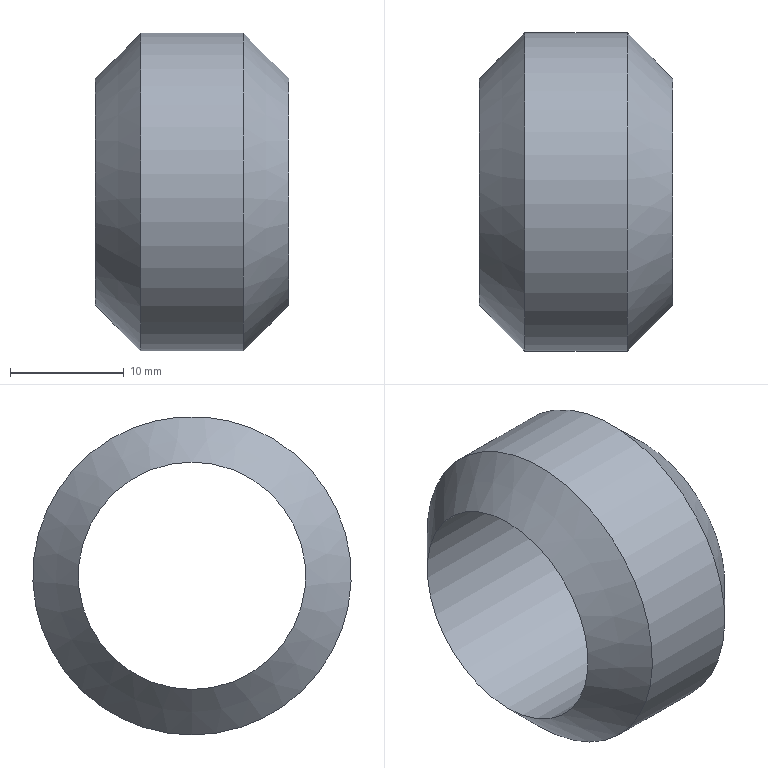Component | NX | PACKING | 1 solid | 4 faces | box 17 x 28 x 28 mm | volume 3854 mm3 | cone 2 | cylinder 2 | commonest cylinder face diameters 28 x1 20 x1
STEP:
#1=CARTESIAN_POINT('',(0.,0.,0.));
#2=DIRECTION('',(0.,0.,1.));
#3=DIRECTION('',(1.,0.,0.));
#4=AXIS2_PLACEMENT_3D('',#1,#2,#3);
#5=CARTESIAN_POINT('',(-29.,0.,-4.5));
#6=VERTEX_POINT('',#5);
#7=CARTESIAN_POINT('',(-29.,0.,9.5));
#8=DIRECTION('',(-1.,0.,0.));
#9=DIRECTION('',(0.,0.,-1.));
#10=AXIS2_PLACEMENT_3D('',#7,#8,#9);
#11=CIRCLE('',#10,14.);
#12=CARTESIAN_POINT('',(-25.,0.,9.5));
#13=DIRECTION('',(-1.,0.,0.));
#14=DIRECTION('',(0.,0.,-1.));
#15=AXIS2_PLACEMENT_3D('',#12,#13,#14);
#16=CONICAL_SURFACE('',#15,10.,0.7854);
#17=CARTESIAN_POINT('',(0.,4.));
#18=DIRECTION('',(1.,0.));
#19=VECTOR('',#18,1.);
#20=LINE('',#17,#19);
#21=(GEOMETRIC_REPRESENTATION_CONTEXT(2)PARAMETRIC_REPRESENTATION_CONTEXT()REPRESENTATION_CONTEXT('',''));
#22=DEFINITIONAL_REPRESENTATION('',(#20),#21);
#23=PCURVE('',#16,#22);
#24=CARTESIAN_POINT('',(-33.5,0.,9.5));
#25=DIRECTION('',(-1.,0.,0.));
#26=DIRECTION('',(0.,0.,-1.));
#27=AXIS2_PLACEMENT_3D('',#24,#25,#26);
#28=CYLINDRICAL_SURFACE('',#27,14.);
#29=CARTESIAN_POINT('',(0.,-4.5));
#30=DIRECTION('',(1.,0.));
#31=VECTOR('',#30,1.);
#32=LINE('',#29,#31);
#33=(GEOMETRIC_REPRESENTATION_CONTEXT(2)PARAMETRIC_REPRESENTATION_CONTEXT()REPRESENTATION_CONTEXT('',''));
#34=DEFINITIONAL_REPRESENTATION('',(#32),#33);
#35=PCURVE('',#28,#34);
#36=SURFACE_CURVE('',#11,(#23,#35),.PCURVE_S1.);
#37=EDGE_CURVE('',#6,#6,#36,.T.);
#38=ORIENTED_EDGE('',*,*,#37,.F.);
#39=CARTESIAN_POINT('',(-25.,0.,-0.5));
#40=VERTEX_POINT('',#39);
#41=CARTESIAN_POINT('',(-25.,0.,-0.5));
#42=CARTESIAN_POINT('',(-29.,0.,-4.5));
#43=B_SPLINE_CURVE_WITH_KNOTS('',1,(#41,#42),.UNSPECIFIED.,.F.,.F.,(2,2),(0.,5.657),.PIECEWISE_BEZIER_KNOTS.);
#44=CARTESIAN_POINT('',(0.,0.));
#45=DIRECTION('',(0.,1.));
#46=VECTOR('',#45,1.);
#47=LINE('',#44,#46);
#48=(GEOMETRIC_REPRESENTATION_CONTEXT(2)PARAMETRIC_REPRESENTATION_CONTEXT()REPRESENTATION_CONTEXT('',''));
#49=DEFINITIONAL_REPRESENTATION('',(#47),#48);
#50=PCURVE('',#16,#49);
#51=CARTESIAN_POINT('',(6.283,0.));
#52=DIRECTION('',(0.,1.));
#53=VECTOR('',#52,1.);
#54=LINE('',#51,#53);
#55=(GEOMETRIC_REPRESENTATION_CONTEXT(2)PARAMETRIC_REPRESENTATION_CONTEXT()REPRESENTATION_CONTEXT('',''));
#56=DEFINITIONAL_REPRESENTATION('',(#54),#55);
#57=PCURVE('',#16,#56);
#58=SEAM_CURVE('',#43,(#50,#57),.PCURVE_S1.);
#59=EDGE_CURVE('',#40,#6,#58,.T.);
#60=ORIENTED_EDGE('',*,*,#59,.F.);
#61=CARTESIAN_POINT('',(-25.,0.,9.5));
#62=DIRECTION('',(-1.,0.,0.));
#63=DIRECTION('',(0.,0.,-1.));
#64=AXIS2_PLACEMENT_3D('',#61,#62,#63);
#65=CIRCLE('',#64,10.);
#66=CARTESIAN_POINT('',(0.,0.));
#67=DIRECTION('',(1.,0.));
#68=VECTOR('',#67,1.);
#69=LINE('',#66,#68);
#70=(GEOMETRIC_REPRESENTATION_CONTEXT(2)PARAMETRIC_REPRESENTATION_CONTEXT()REPRESENTATION_CONTEXT('',''));
#71=DEFINITIONAL_REPRESENTATION('',(#69),#70);
#72=PCURVE('',#16,#71);
#73=CARTESIAN_POINT('',(-33.5,0.,9.5));
#74=DIRECTION('',(-1.,0.,0.));
#75=DIRECTION('',(0.,0.,-1.));
#76=AXIS2_PLACEMENT_3D('',#73,#74,#75);
#77=CYLINDRICAL_SURFACE('',#76,10.);
#78=CARTESIAN_POINT('',(0.,-8.5));
#79=DIRECTION('',(1.,0.));
#80=VECTOR('',#79,1.);
#81=LINE('',#78,#80);
#82=(GEOMETRIC_REPRESENTATION_CONTEXT(2)PARAMETRIC_REPRESENTATION_CONTEXT()REPRESENTATION_CONTEXT('',''));
#83=DEFINITIONAL_REPRESENTATION('',(#81),#82);
#84=PCURVE('',#77,#83);
#85=SURFACE_CURVE('',#65,(#72,#84),.PCURVE_S1.);
#86=EDGE_CURVE('',#40,#40,#85,.T.);
#87=ORIENTED_EDGE('',*,*,#86,.T.);
#88=ORIENTED_EDGE('',*,*,#59,.T.);
#89=EDGE_LOOP('',(#38,#60,#87,#88));
#90=FACE_BOUND('',#89,.T.);
#91=ADVANCED_FACE('',(#90),#16,.T.);
#92=CARTESIAN_POINT('',(-38.,0.,-4.5));
#93=VERTEX_POINT('',#92);
#94=CARTESIAN_POINT('',(-38.,0.,9.5));
#95=DIRECTION('',(-1.,0.,0.));
#96=DIRECTION('',(0.,0.,-1.));
#97=AXIS2_PLACEMENT_3D('',#94,#95,#96);
#98=CIRCLE('',#97,14.);
#99=CARTESIAN_POINT('',(0.,4.5));
#100=DIRECTION('',(1.,0.));
#101=VECTOR('',#100,1.);
#102=LINE('',#99,#101);
#103=(GEOMETRIC_REPRESENTATION_CONTEXT(2)PARAMETRIC_REPRESENTATION_CONTEXT()REPRESENTATION_CONTEXT('',''));
#104=DEFINITIONAL_REPRESENTATION('',(#102),#103);
#105=PCURVE('',#28,#104);
#106=CARTESIAN_POINT('',(-38.,0.,9.5));
#107=DIRECTION('',(1.,0.,0.));
#108=DIRECTION('',(0.,0.,1.));
#109=AXIS2_PLACEMENT_3D('',#106,#107,#108);
#110=CONICAL_SURFACE('',#109,14.,0.7854);
#111=CARTESIAN_POINT('',(9.425,0.));
#112=DIRECTION('',(-1.,0.));
#113=VECTOR('',#112,1.);
#114=LINE('',#111,#113);
#115=(GEOMETRIC_REPRESENTATION_CONTEXT(2)PARAMETRIC_REPRESENTATION_CONTEXT()REPRESENTATION_CONTEXT('',''));
#116=DEFINITIONAL_REPRESENTATION('',(#114),#115);
#117=PCURVE('',#110,#116);
#118=SURFACE_CURVE('',#98,(#105,#117),.PCURVE_S1.);
#119=EDGE_CURVE('',#93,#93,#118,.T.);
#120=ORIENTED_EDGE('',*,*,#119,.F.);
#121=CARTESIAN_POINT('',(-29.,0.,-4.5));
#122=CARTESIAN_POINT('',(-38.,0.,-4.5));
#123=B_SPLINE_CURVE_WITH_KNOTS('',1,(#121,#122),.UNSPECIFIED.,.F.,.F.,(2,2),(-4.5,4.5),.PIECEWISE_BEZIER_KNOTS.);
#124=CARTESIAN_POINT('',(0.,0.));
#125=DIRECTION('',(0.,1.));
#126=VECTOR('',#125,1.);
#127=LINE('',#124,#126);
#128=(GEOMETRIC_REPRESENTATION_CONTEXT(2)PARAMETRIC_REPRESENTATION_CONTEXT()REPRESENTATION_CONTEXT('',''));
#129=DEFINITIONAL_REPRESENTATION('',(#127),#128);
#130=PCURVE('',#28,#129);
#131=CARTESIAN_POINT('',(6.283,0.));
#132=DIRECTION('',(0.,1.));
#133=VECTOR('',#132,1.);
#134=LINE('',#131,#133);
#135=(GEOMETRIC_REPRESENTATION_CONTEXT(2)PARAMETRIC_REPRESENTATION_CONTEXT()REPRESENTATION_CONTEXT('',''));
#136=DEFINITIONAL_REPRESENTATION('',(#134),#135);
#137=PCURVE('',#28,#136);
#138=SEAM_CURVE('',#123,(#130,#137),.PCURVE_S1.);
#139=EDGE_CURVE('',#6,#93,#138,.T.);
#140=ORIENTED_EDGE('',*,*,#139,.F.);
#141=ORIENTED_EDGE('',*,*,#37,.T.);
#142=ORIENTED_EDGE('',*,*,#139,.T.);
#143=EDGE_LOOP('',(#120,#140,#141,#142));
#144=FACE_BOUND('',#143,.T.);
#145=ADVANCED_FACE('',(#144),#28,.T.);
#146=CARTESIAN_POINT('',(-42.,0.,-0.5));
#147=VERTEX_POINT('',#146);
#148=CARTESIAN_POINT('',(-42.,0.,9.5));
#149=DIRECTION('',(-1.,0.,0.));
#150=DIRECTION('',(0.,0.,-1.));
#151=AXIS2_PLACEMENT_3D('',#148,#149,#150);
#152=CIRCLE('',#151,10.);
#153=CARTESIAN_POINT('',(9.425,-4.));
#154=DIRECTION('',(-1.,0.));
#155=VECTOR('',#154,1.);
#156=LINE('',#153,#155);
#157=(GEOMETRIC_REPRESENTATION_CONTEXT(2)PARAMETRIC_REPRESENTATION_CONTEXT()REPRESENTATION_CONTEXT('',''));
#158=DEFINITIONAL_REPRESENTATION('',(#156),#157);
#159=PCURVE('',#110,#158);
#160=CARTESIAN_POINT('',(0.,8.5));
#161=DIRECTION('',(1.,0.));
#162=VECTOR('',#161,1.);
#163=LINE('',#160,#162);
#164=(GEOMETRIC_REPRESENTATION_CONTEXT(2)PARAMETRIC_REPRESENTATION_CONTEXT()REPRESENTATION_CONTEXT('',''));
#165=DEFINITIONAL_REPRESENTATION('',(#163),#164);
#166=PCURVE('',#77,#165);
#167=SURFACE_CURVE('',#152,(#159,#166),.PCURVE_S1.);
#168=EDGE_CURVE('',#147,#147,#167,.T.);
#169=ORIENTED_EDGE('',*,*,#168,.F.);
#170=CARTESIAN_POINT('',(-42.,0.,-0.5));
#171=CARTESIAN_POINT('',(-38.,0.,-4.5));
#172=B_SPLINE_CURVE_WITH_KNOTS('',1,(#170,#171),.UNSPECIFIED.,.F.,.F.,(2,2),(-5.657,0.),.PIECEWISE_BEZIER_KNOTS.);
#173=CARTESIAN_POINT('',(9.425,0.));
#174=DIRECTION('',(0.,1.));
#175=VECTOR('',#174,1.);
#176=LINE('',#173,#175);
#177=(GEOMETRIC_REPRESENTATION_CONTEXT(2)PARAMETRIC_REPRESENTATION_CONTEXT()REPRESENTATION_CONTEXT('',''));
#178=DEFINITIONAL_REPRESENTATION('',(#176),#177);
#179=PCURVE('',#110,#178);
#180=CARTESIAN_POINT('',(3.142,0.));
#181=DIRECTION('',(0.,1.));
#182=VECTOR('',#181,1.);
#183=LINE('',#180,#182);
#184=(GEOMETRIC_REPRESENTATION_CONTEXT(2)PARAMETRIC_REPRESENTATION_CONTEXT()REPRESENTATION_CONTEXT('',''));
#185=DEFINITIONAL_REPRESENTATION('',(#183),#184);
#186=PCURVE('',#110,#185);
#187=SEAM_CURVE('',#172,(#179,#186),.PCURVE_S1.);
#188=EDGE_CURVE('',#147,#93,#187,.T.);
#189=ORIENTED_EDGE('',*,*,#188,.T.);
#190=ORIENTED_EDGE('',*,*,#119,.T.);
#191=ORIENTED_EDGE('',*,*,#188,.F.);
#192=EDGE_LOOP('',(#169,#189,#190,#191));
#193=FACE_BOUND('',#192,.T.);
#194=ADVANCED_FACE('',(#193),#110,.T.);
#195=ORIENTED_EDGE('',*,*,#86,.T.);
#196=CARTESIAN_POINT('',(-25.,0.,-0.5));
#197=CARTESIAN_POINT('',(-42.,0.,-0.5));
#198=B_SPLINE_CURVE_WITH_KNOTS('',1,(#196,#197),.UNSPECIFIED.,.F.,.F.,(2,2),(-8.5,8.5),.PIECEWISE_BEZIER_KNOTS.);
#199=CARTESIAN_POINT('',(6.283,0.));
#200=DIRECTION('',(0.,1.));
#201=VECTOR('',#200,1.);
#202=LINE('',#199,#201);
#203=(GEOMETRIC_REPRESENTATION_CONTEXT(2)PARAMETRIC_REPRESENTATION_CONTEXT()REPRESENTATION_CONTEXT('',''));
#204=DEFINITIONAL_REPRESENTATION('',(#202),#203);
#205=PCURVE('',#77,#204);
#206=CARTESIAN_POINT('',(0.,0.));
#207=DIRECTION('',(0.,1.));
#208=VECTOR('',#207,1.);
#209=LINE('',#206,#208);
#210=(GEOMETRIC_REPRESENTATION_CONTEXT(2)PARAMETRIC_REPRESENTATION_CONTEXT()REPRESENTATION_CONTEXT('',''));
#211=DEFINITIONAL_REPRESENTATION('',(#209),#210);
#212=PCURVE('',#77,#211);
#213=SEAM_CURVE('',#198,(#205,#212),.PCURVE_S1.);
#214=EDGE_CURVE('',#40,#147,#213,.T.);
#215=ORIENTED_EDGE('',*,*,#214,.T.);
#216=ORIENTED_EDGE('',*,*,#168,.F.);
#217=ORIENTED_EDGE('',*,*,#214,.F.);
#218=EDGE_LOOP('',(#195,#215,#216,#217));
#219=FACE_BOUND('',#218,.F.);
#220=ADVANCED_FACE('',(#219),#77,.F.);
#221=CLOSED_SHELL('',(#91,#145,#194,#220));
#222=MANIFOLD_SOLID_BREP('',#221);
#223=(LENGTH_UNIT()NAMED_UNIT(*)SI_UNIT(.MILLI.,.METRE.));
#224=UNCERTAINTY_MEASURE_WITH_UNIT(LENGTH_MEASURE(0.00001),#223,'','');
#225=(NAMED_UNIT(*)PLANE_ANGLE_UNIT()SI_UNIT($,.RADIAN.));
#226=(NAMED_UNIT(*)SI_UNIT($,.STERADIAN.)SOLID_ANGLE_UNIT());
#227=(GEOMETRIC_REPRESENTATION_CONTEXT(3)GLOBAL_UNCERTAINTY_ASSIGNED_CONTEXT((#224))GLOBAL_UNIT_ASSIGNED_CONTEXT((#223,#225,#226))REPRESENTATION_CONTEXT('',''));
#228=ADVANCED_BREP_SHAPE_REPRESENTATION('',(#4,#222),#227);